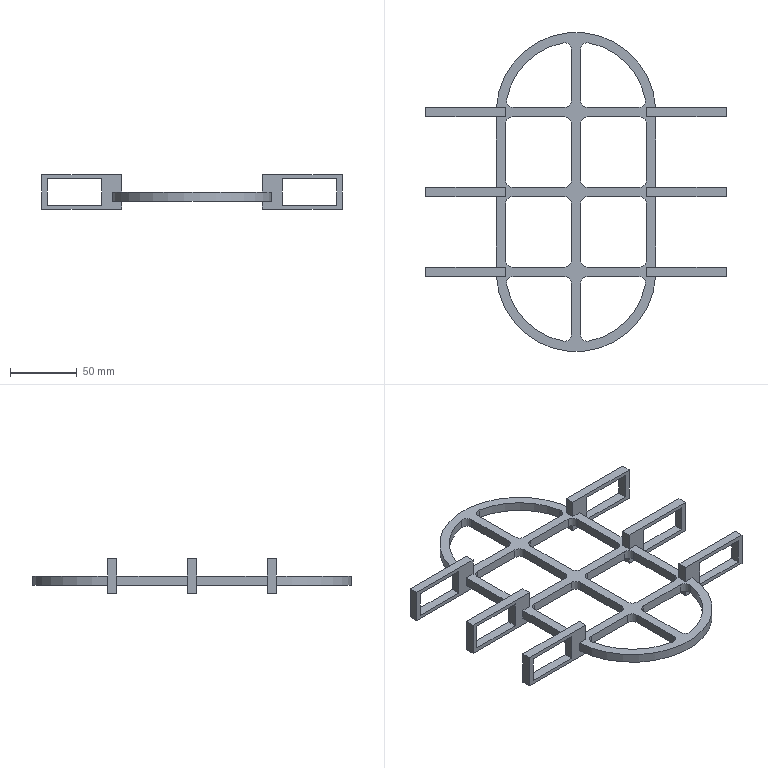Component | NX | BOTTOM_COVER | 1 solid | 130 faces | volume 84964 mm3 | plane 96 | cylinder 34 | commonest cylinder face diameters 10 x28 106 x4 120 x2